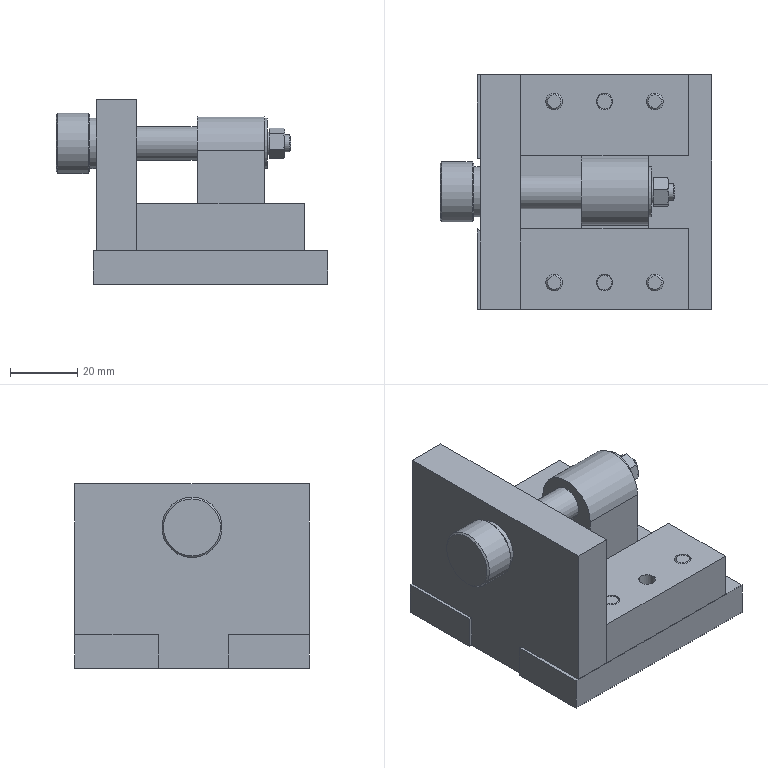Assembly | NX | mm | 16 component files | 16 solids | 242 faces | box 81 x 70 x 55 mm | volume 133542 mm3 | plane 134 | cone 56 | cylinder 44 | torus 8 | commonest cylinder face diameters 5 x14 4.826 x8 10 x6 8.5 x4 5.5 x4 15 x2 8 x2 6.9 x1
Bill of materials:
unnamed part 1 | 1 |  | Flat rectangular plate with one round through hole near the top edge and a rectangular tab sticking out from the bottom edge, set slightly left of center.
unnamed part 2 | 1 |  | Solid turned stepped shaft or pin: a larger cylindrical head with chamfered edges, a short collar step, then three cylindrical sections that get smaller toward a chamfered tip.
unnamed part 3 | 4 |  | Plain solid cylindrical pin with chamfers at both ends.
GB-T6170_T-2000,M5x0.8 | 1 |  | Hexagonal prism with a central round through bore, chamfered hex corners on one face, and a short cylindrical collar on the other face, giving it a hex-nut-like shape.
GB-T96_1-2002,M5 | 1 |  | Thin, flat annular disk (a plain ring shape) with one concentric circular through-hole and flat, parallel faces. Its shape is consistent with a plain flat washer.
unnamed part 4 | 1 |  | Bracket with a rectangular base block and a centered upright lug with a semicircular top and a horizontal round through hole, forming an inverted-T profile.
GB-T70.1-2000,M5x20 | 4 |  | Hexagon Socket Head Cap Screw, GB-T 70.1-2000,M5x20
unnamed part 5 | 1 |  | Flat, roughly square plate with eight round through holes in two rows of four along opposite edges, and a notch cut into one side edge with one square corner and one angled edge.
unnamed part 6 | 2 |  | Rectangular bar or block with an L-shaped (stepped/rebated) cross-section running its full length, and three round through holes evenly spaced in a row along the length.
Mates:
1. fix | base_plate 1 component
2. touch align | cylinder_shaft 1 face | T_slider 1 face
3. touch align | cylinder_shaft 1 face | T_slider 1 face
4. touch align | T_slider 1 face | base_plate 1 face
5. touch align | guide_plate 2 face | base_plate 1 face
6. touch align | guide_plate 2 face | base_plate 1 face
7. parallel | guide_plate 2 face | base_plate 1 face
8. touch align | T_slider 1 face | guide_plate 2 face
9. touch align | support_plate 1 face | cylinder_shaft 1 face
10. touch align | support_plate 1 face | base_plate 1 face
11. touch align | cylinder_shaft 1 face | support_plate 1 face
12. touch align | dowel_pin_5x20 4 face | guide_plate 2 face
13. touch align | dowel_pin_5x20 3 face | guide_plate 2 face
14. touch align | dowel_pin_5x20 3 face | guide_plate 2 face
15. touch align | dowel_pin_5x20 4 face | guide_plate 2 face
16. touch align | GB-T96_1-2002_M5 1 face | T_slider 1 face
17. touch align | GB-T6170_T-2000_M5x0_8 1 face | GB-T96_1-2002_M5 1 face
18. touch align | GB-T70_1-2000_M5x15 4 face | base_plate 1 face
19. touch align | GB-T70_1-2000_M5x15 4 face | base_plate 1 face
20. touch align | GB-T70_1-2000_M5x15 3 face | base_plate 1 face
21. touch align | GB-T70_1-2000_M5x15 3 face | base_plate 1 face